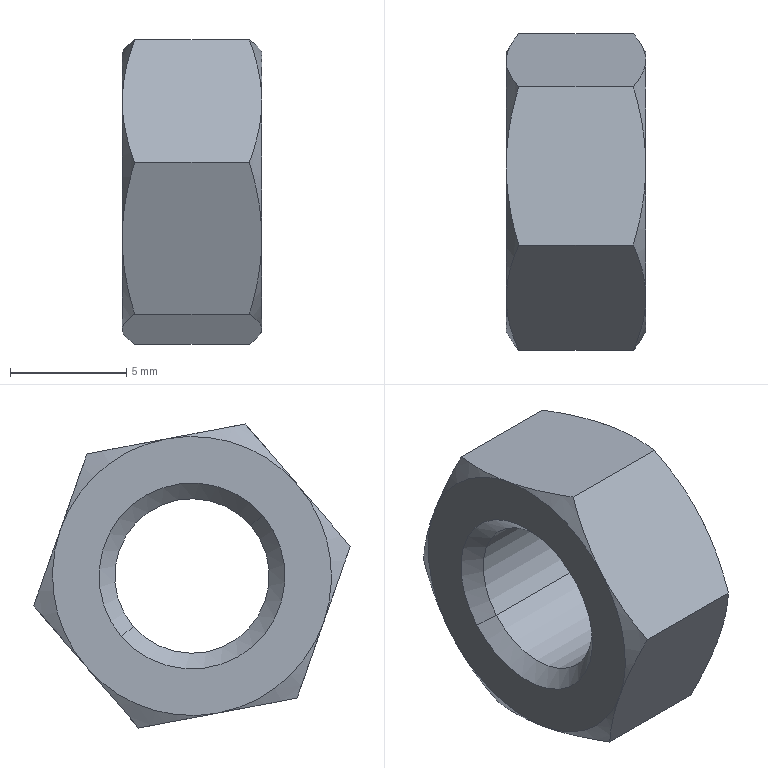Component | SolidWorks | CCDJSMA20x160SU(0)+(CS1-M-2)-1_CCDJS20 MA Nut1-1 | 1 solid | 26 faces | box 6 x 13.62 x 13.08 mm | volume 526 mm3 | cone 16 | plane 8 | cylinder 2 | commonest cylinder face diameters 6.647 x2
build123d program:
from build123d import *

# Parameters (mm, degrees)
CUT_EXTRUDE1_DEPTH      = 3
CUT_EXTRUDE1_DEPTH_BACK = 3
SKETCH3_W               = 24
SKETCH3_H               = 24


with BuildPart() as part:
    # Sketch1 → Revolve1 (revolve)
    with BuildSketch(Plane.XY, mode=Mode.PRIVATE) as revolve1_sk:
        Polygon((-3, 0), (-3, 6), (-2.307, 7.2), (2.307, 7.2), (3, 6), (3, 0), align=None)
    revolve(revolve1_sk.sketch.rotate(Axis((3, 0, 0), (-1, 0, 0)), 270), axis=Axis((3, 0, 0), (-1, 0, 0)))

    # Sketch2 → Cut-Revolve1 (revolve, cut)
    with BuildSketch(Plane.XY, mode=Mode.PRIVATE) as cut_revolve1_sk:
        Polygon((-3, 0), (-3, 4), (-2.324, 3.324), (2.324, 3.324), (3, 4), (3, 0), align=None)
    revolve(cut_revolve1_sk.sketch.rotate(Axis((3, 0, 0), (-1, 0, 0)), 270), axis=Axis((3, 0, 0), (-1, 0, 0)), mode=Mode.SUBTRACT)

    # Sketch3 → Cut-Extrude1 (cut, two sides: drawn at the far end of the back side and taken through both)
    with BuildSketch(Plane(origin=(0, 0, 0), x_dir=(0, 0, -1), z_dir=(1, 0, 0)).offset(-CUT_EXTRUDE1_DEPTH_BACK)):
        Rectangle(SKETCH3_W, SKETCH3_H)
        Polygon((-6, -3.464), (0, -6.928), (6, -3.464), (6, 3.464), (0, 6.928), (-6, 3.464), align=None, mode=Mode.SUBTRACT)
    extrude(amount=CUT_EXTRUDE1_DEPTH + CUT_EXTRUDE1_DEPTH_BACK, mode=Mode.SUBTRACT)


solid = part.part

# Placed as in the assembly
solid = solid.moved(Location((-82, 426.564, -63.57), (49.332, 0, 180)))
STEP:
#1=CARTESIAN_POINT('',(-3.32,16.695,-2.417));
#2=VERTEX_POINT('',#1);
#3=CARTESIAN_POINT('',(-3.32,16.893,-2.588));
#4=VERTEX_POINT('',#3);
#5=CARTESIAN_POINT('',(-3.32,16.794,-2.503));
#6=DIRECTION('',(1.,0.,0.));
#7=DIRECTION('',(0.,0.7584,-0.6518));
#8=AXIS2_PLACEMENT_3D('',#5,#6,#7);
#9=CIRCLE('',#8,0.1308);
#10=EDGE_CURVE('',#2,#4,#9,.T.);
#11=ORIENTED_EDGE('',*,*,#10,.T.);
#12=CARTESIAN_POINT('',(-3.346,16.913,-2.605));
#13=VERTEX_POINT('',#12);
#14=CARTESIAN_POINT('',(-3.346,16.913,-2.605));
#15=DIRECTION('',(-0.7071,0.5363,-0.4609));
#16=VECTOR('',#15,39.37);
#17=LINE('',#14,#16);
#18=EDGE_CURVE('',#4,#13,#17,.T.);
#19=ORIENTED_EDGE('',*,*,#18,.T.);
#20=CARTESIAN_POINT('',(-3.346,16.674,-2.4));
#21=VERTEX_POINT('',#20);
#22=CARTESIAN_POINT('',(-3.346,16.794,-2.503));
#23=DIRECTION('',(1.,0.,0.));
#24=DIRECTION('',(0.,0.7584,-0.6518));
#25=AXIS2_PLACEMENT_3D('',#22,#23,#24);
#26=CIRCLE('',#25,0.1575);
#27=EDGE_CURVE('',#21,#13,#26,.T.);
#28=ORIENTED_EDGE('',*,*,#27,.F.);
#29=CARTESIAN_POINT('',(-3.346,16.674,-2.4));
#30=DIRECTION('',(-0.7071,-0.5363,0.4609));
#31=VECTOR('',#30,39.37);
#32=LINE('',#29,#31);
#33=EDGE_CURVE('',#2,#21,#32,.T.);
#34=ORIENTED_EDGE('',*,*,#33,.F.);
#35=EDGE_LOOP('',(#11,#19,#28,#34));
#36=FACE_OUTER_BOUND('',#35,.T.);
#37=CARTESIAN_POINT('',(-3.346,16.794,-2.503));
#38=DIRECTION('',(-1.,0.,0.));
#39=DIRECTION('',(0.,-0.7584,0.6518));
#40=AXIS2_PLACEMENT_3D('',#37,#38,#39);
#41=CONICAL_SURFACE('',#40,0.1575,0.7854);
#42=ADVANCED_FACE('',(#36),#41,.F.);
#43=ORIENTED_EDGE('',*,*,#10,.F.);
#44=CARTESIAN_POINT('',(-3.137,16.695,-2.417));
#45=VERTEX_POINT('',#44);
#46=CARTESIAN_POINT('',(-3.346,16.695,-2.417));
#47=DIRECTION('',(1.,0.,0.));
#48=VECTOR('',#47,39.37);
#49=LINE('',#46,#48);
#50=EDGE_CURVE('',#2,#45,#49,.T.);
#51=ORIENTED_EDGE('',*,*,#50,.T.);
#52=CARTESIAN_POINT('',(-3.137,16.893,-2.588));
#53=VERTEX_POINT('',#52);
#54=CARTESIAN_POINT('',(-3.137,16.794,-2.503));
#55=DIRECTION('',(1.,0.,0.));
#56=DIRECTION('',(0.,0.7584,-0.6518));
#57=AXIS2_PLACEMENT_3D('',#54,#55,#56);
#58=CIRCLE('',#57,0.1308);
#59=EDGE_CURVE('',#45,#53,#58,.T.);
#60=ORIENTED_EDGE('',*,*,#59,.T.);
#61=CARTESIAN_POINT('',(-3.346,16.893,-2.588));
#62=DIRECTION('',(1.,0.,0.));
#63=VECTOR('',#62,39.37);
#64=LINE('',#61,#63);
#65=EDGE_CURVE('',#4,#53,#64,.T.);
#66=ORIENTED_EDGE('',*,*,#65,.F.);
#67=EDGE_LOOP('',(#43,#51,#60,#66));
#68=FACE_OUTER_BOUND('',#67,.T.);
#69=CARTESIAN_POINT('',(-3.346,16.794,-2.503));
#70=DIRECTION('',(1.,0.,0.));
#71=DIRECTION('',(0.,0.7584,-0.6518));
#72=AXIS2_PLACEMENT_3D('',#69,#70,#71);
#73=CYLINDRICAL_SURFACE('',#72,0.1308);
#74=ADVANCED_FACE('',(#68),#73,.F.);
#75=ORIENTED_EDGE('',*,*,#59,.F.);
#76=CARTESIAN_POINT('',(-3.11,16.674,-2.4));
#77=VERTEX_POINT('',#76);
#78=CARTESIAN_POINT('',(-3.137,16.695,-2.417));
#79=DIRECTION('',(0.7071,-0.5363,0.4609));
#80=VECTOR('',#79,39.37);
#81=LINE('',#78,#80);
#82=EDGE_CURVE('',#45,#77,#81,.T.);
#83=ORIENTED_EDGE('',*,*,#82,.T.);
#84=CARTESIAN_POINT('',(-3.11,16.913,-2.605));
#85=VERTEX_POINT('',#84);
#86=CARTESIAN_POINT('',(-3.11,16.794,-2.503));
#87=DIRECTION('',(1.,0.,0.));
#88=DIRECTION('',(0.,0.7584,-0.6518));
#89=AXIS2_PLACEMENT_3D('',#86,#87,#88);
#90=CIRCLE('',#89,0.1575);
#91=EDGE_CURVE('',#77,#85,#90,.T.);
#92=ORIENTED_EDGE('',*,*,#91,.T.);
#93=CARTESIAN_POINT('',(-3.137,16.893,-2.588));
#94=DIRECTION('',(0.7071,0.5363,-0.4609));
#95=VECTOR('',#94,39.37);
#96=LINE('',#93,#95);
#97=EDGE_CURVE('',#53,#85,#96,.T.);
#98=ORIENTED_EDGE('',*,*,#97,.F.);
#99=EDGE_LOOP('',(#75,#83,#92,#98));
#100=FACE_OUTER_BOUND('',#99,.T.);
#101=CARTESIAN_POINT('',(-3.137,16.794,-2.503));
#102=DIRECTION('',(1.,0.,0.));
#103=DIRECTION('',(0.,0.7584,-0.6518));
#104=AXIS2_PLACEMENT_3D('',#101,#102,#103);
#105=CONICAL_SURFACE('',#104,0.1308,0.7854);
#106=ADVANCED_FACE('',(#100),#105,.F.);
#107=CARTESIAN_POINT('',(-3.131,16.704,-2.245));
#108=VERTEX_POINT('',#107);
#109=CARTESIAN_POINT('',(-3.11,16.838,-2.271));
#110=VERTEX_POINT('',#109);
#111=CARTESIAN_POINT('',(-3.131,16.704,-2.245));
#112=CARTESIAN_POINT('',(-3.118,16.747,-2.254));
#113=CARTESIAN_POINT('',(-3.11,16.792,-2.262));
#114=CARTESIAN_POINT('',(-3.11,16.838,-2.271));
#115=B_SPLINE_CURVE_WITH_KNOTS('',3,(#111,#112,#113,#114),.UNSPECIFIED.,.F.,.F.,(4,4),(0.00000024,0.003505),.UNSPECIFIED.);
#116=EDGE_CURVE('',#108,#110,#115,.T.);
#117=ORIENTED_EDGE('',*,*,#116,.F.);
#118=CARTESIAN_POINT('',(-3.11,16.615,-2.349));
#119=VERTEX_POINT('',#118);
#120=CARTESIAN_POINT('',(-3.11,16.615,-2.349));
#121=CARTESIAN_POINT('',(-3.11,16.63,-2.331));
#122=CARTESIAN_POINT('',(-3.112,16.645,-2.314));
#123=CARTESIAN_POINT('',(-3.12,16.675,-2.279));
#124=CARTESIAN_POINT('',(-3.125,16.689,-2.262));
#125=CARTESIAN_POINT('',(-3.131,16.704,-2.245));
#126=B_SPLINE_CURVE_WITH_KNOTS('',3,(#120,#121,#122,#123,#124,#125),.UNSPECIFIED.,.F.,.F.,(4,2,4),(0.009709,0.01146,0.01322),.UNSPECIFIED.);
#127=EDGE_CURVE('',#119,#108,#126,.T.);
#128=ORIENTED_EDGE('',*,*,#127,.F.);
#129=CARTESIAN_POINT('',(-3.11,16.794,-2.503));
#130=DIRECTION('',(1.,0.,0.));
#131=DIRECTION('',(0.,0.7584,-0.6518));
#132=AXIS2_PLACEMENT_3D('',#129,#130,#131);
#133=CIRCLE('',#132,0.2362);
#134=EDGE_CURVE('',#110,#119,#133,.T.);
#135=ORIENTED_EDGE('',*,*,#134,.F.);
#136=EDGE_LOOP('',(#117,#128,#135));
#137=FACE_OUTER_BOUND('',#136,.T.);
#138=CARTESIAN_POINT('',(-3.138,16.794,-2.503));
#139=DIRECTION('',(-1.,0.,0.));
#140=DIRECTION('',(0.,-0.7584,0.6518));
#141=AXIS2_PLACEMENT_3D('',#138,#139,#140);
#142=CONICAL_SURFACE('',#141,0.2835,1.047);
#143=ADVANCED_FACE('',(#137),#142,.T.);
#144=CARTESIAN_POINT('',(-3.131,16.972,-2.296));
#145=VERTEX_POINT('',#144);
#146=CARTESIAN_POINT('',(-3.11,16.838,-2.271));
#147=CARTESIAN_POINT('',(-3.11,16.849,-2.273));
#148=CARTESIAN_POINT('',(-3.111,16.86,-2.275));
#149=CARTESIAN_POINT('',(-3.113,16.883,-2.279));
#150=CARTESIAN_POINT('',(-3.114,16.894,-2.281));
#151=CARTESIAN_POINT('',(-3.12,16.928,-2.288));
#152=CARTESIAN_POINT('',(-3.125,16.95,-2.292));
#153=CARTESIAN_POINT('',(-3.131,16.972,-2.296));
#154=B_SPLINE_CURVE_WITH_KNOTS('',3,(#146,#147,#148,#149,#150,#151,#152,#153),.UNSPECIFIED.,.F.,.F.,(4,2,2,4),(0.003505,0.004378,0.005251,0.006997),.UNSPECIFIED.);
#155=EDGE_CURVE('',#110,#145,#154,.T.);
#156=ORIENTED_EDGE('',*,*,#155,.F.);
#157=CARTESIAN_POINT('',(-3.11,17.017,-2.425));
#158=VERTEX_POINT('',#157);
#159=CARTESIAN_POINT('',(-3.11,16.794,-2.503));
#160=DIRECTION('',(1.,0.,0.));
#161=DIRECTION('',(0.,0.7584,-0.6518));
#162=AXIS2_PLACEMENT_3D('',#159,#160,#161);
#163=CIRCLE('',#162,0.2362);
#164=EDGE_CURVE('',#158,#110,#163,.T.);
#165=ORIENTED_EDGE('',*,*,#164,.F.);
#166=CARTESIAN_POINT('',(-3.131,16.972,-2.296));
#167=CARTESIAN_POINT('',(-3.118,16.986,-2.338));
#168=CARTESIAN_POINT('',(-3.11,17.001,-2.381));
#169=CARTESIAN_POINT('',(-3.11,17.017,-2.425));
#170=B_SPLINE_CURVE_WITH_KNOTS('',3,(#166,#167,#168,#169),.UNSPECIFIED.,.F.,.F.,(4,4),(0.00000024,0.003505),.UNSPECIFIED.);
#171=EDGE_CURVE('',#145,#158,#170,.T.);
#172=ORIENTED_EDGE('',*,*,#171,.F.);
#173=EDGE_LOOP('',(#156,#165,#172));
#174=FACE_OUTER_BOUND('',#173,.T.);
#175=CARTESIAN_POINT('',(-3.138,16.794,-2.503));
#176=DIRECTION('',(-1.,0.,0.));
#177=DIRECTION('',(0.,-0.7584,0.6518));
#178=AXIS2_PLACEMENT_3D('',#175,#176,#177);
#179=CONICAL_SURFACE('',#178,0.2835,1.047);
#180=ADVANCED_FACE('',(#174),#179,.T.);
#181=CARTESIAN_POINT('',(-3.131,17.062,-2.553));
#182=VERTEX_POINT('',#181);
#183=CARTESIAN_POINT('',(-3.11,17.017,-2.425));
#184=CARTESIAN_POINT('',(-3.11,17.021,-2.436));
#185=CARTESIAN_POINT('',(-3.111,17.024,-2.446));
#186=CARTESIAN_POINT('',(-3.113,17.032,-2.468));
#187=CARTESIAN_POINT('',(-3.114,17.036,-2.479));
#188=CARTESIAN_POINT('',(-3.12,17.047,-2.511));
#189=CARTESIAN_POINT('',(-3.125,17.055,-2.532));
#190=CARTESIAN_POINT('',(-3.131,17.062,-2.553));
#191=B_SPLINE_CURVE_WITH_KNOTS('',3,(#183,#184,#185,#186,#187,#188,#189,#190),.UNSPECIFIED.,.F.,.F.,(4,2,2,4),(0.003505,0.004378,0.005251,0.006997),.UNSPECIFIED.);
#192=EDGE_CURVE('',#158,#182,#191,.T.);
#193=ORIENTED_EDGE('',*,*,#192,.F.);
#194=CARTESIAN_POINT('',(-3.11,16.973,-2.657));
#195=VERTEX_POINT('',#194);
#196=CARTESIAN_POINT('',(-3.11,16.794,-2.503));
#197=DIRECTION('',(1.,0.,0.));
#198=DIRECTION('',(0.,0.7584,-0.6518));
#199=AXIS2_PLACEMENT_3D('',#196,#197,#198);
#200=CIRCLE('',#199,0.2362);
#201=EDGE_CURVE('',#195,#158,#200,.T.);
#202=ORIENTED_EDGE('',*,*,#201,.F.);
#203=CARTESIAN_POINT('',(-3.131,17.062,-2.553));
#204=CARTESIAN_POINT('',(-3.125,17.048,-2.57));
#205=CARTESIAN_POINT('',(-3.12,17.033,-2.587));
#206=CARTESIAN_POINT('',(-3.112,17.003,-2.622));
#207=CARTESIAN_POINT('',(-3.11,16.988,-2.639));
#208=CARTESIAN_POINT('',(-3.11,16.973,-2.657));
#209=B_SPLINE_CURVE_WITH_KNOTS('',3,(#203,#204,#205,#206,#207,#208),.UNSPECIFIED.,.F.,.F.,(4,2,4),(0.01521,0.01696,0.01872),.UNSPECIFIED.);
#210=EDGE_CURVE('',#182,#195,#209,.T.);
#211=ORIENTED_EDGE('',*,*,#210,.F.);
#212=EDGE_LOOP('',(#193,#202,#211));
#213=FACE_OUTER_BOUND('',#212,.T.);
#214=CARTESIAN_POINT('',(-3.138,16.794,-2.503));
#215=DIRECTION('',(-1.,0.,0.));
#216=DIRECTION('',(0.,-0.7584,0.6518));
#217=AXIS2_PLACEMENT_3D('',#214,#215,#216);
#218=CONICAL_SURFACE('',#217,0.2835,1.047);
#219=ADVANCED_FACE('',(#213),#218,.T.);
#220=CARTESIAN_POINT('',(-3.131,16.526,-2.452));
#221=VERTEX_POINT('',#220);
#222=CARTESIAN_POINT('',(-3.131,16.526,-2.452));
#223=CARTESIAN_POINT('',(-3.125,16.54,-2.435));
#224=CARTESIAN_POINT('',(-3.12,16.555,-2.418));
#225=CARTESIAN_POINT('',(-3.112,16.585,-2.384));
#226=CARTESIAN_POINT('',(-3.11,16.6,-2.366));
#227=CARTESIAN_POINT('',(-3.11,16.615,-2.349));
#228=B_SPLINE_CURVE_WITH_KNOTS('',3,(#222,#223,#224,#225,#226,#227),.UNSPECIFIED.,.F.,.F.,(4,2,4),(0.006205,0.007957,0.009709),.UNSPECIFIED.);
#229=EDGE_CURVE('',#221,#119,#228,.T.);
#230=ORIENTED_EDGE('',*,*,#229,.F.);
#231=CARTESIAN_POINT('',(-3.11,16.571,-2.581));
#232=VERTEX_POINT('',#231);
#233=CARTESIAN_POINT('',(-3.11,16.571,-2.581));
#234=CARTESIAN_POINT('',(-3.11,16.567,-2.57));
#235=CARTESIAN_POINT('',(-3.111,16.563,-2.559));
#236=CARTESIAN_POINT('',(-3.113,16.556,-2.537));
#237=CARTESIAN_POINT('',(-3.114,16.552,-2.527));
#238=CARTESIAN_POINT('',(-3.12,16.541,-2.494));
#239=CARTESIAN_POINT('',(-3.125,16.533,-2.473));
#240=CARTESIAN_POINT('',(-3.131,16.526,-2.452));
#241=B_SPLINE_CURVE_WITH_KNOTS('',3,(#233,#234,#235,#236,#237,#238,#239,#240),.UNSPECIFIED.,.F.,.F.,(4,2,2,4),(0.003505,0.004378,0.005251,0.006997),.UNSPECIFIED.);
#242=EDGE_CURVE('',#232,#221,#241,.T.);
#243=ORIENTED_EDGE('',*,*,#242,.F.);
#244=CARTESIAN_POINT('',(-3.11,16.794,-2.503));
#245=DIRECTION('',(1.,0.,0.));
#246=DIRECTION('',(0.,0.7584,-0.6518));
#247=AXIS2_PLACEMENT_3D('',#244,#245,#246);
#248=CIRCLE('',#247,0.2362);
#249=EDGE_CURVE('',#119,#232,#248,.T.);
#250=ORIENTED_EDGE('',*,*,#249,.F.);
#251=EDGE_LOOP('',(#230,#243,#250));
#252=FACE_OUTER_BOUND('',#251,.T.);
#253=CARTESIAN_POINT('',(-3.138,16.794,-2.503));
#254=DIRECTION('',(-1.,0.,0.));
#255=DIRECTION('',(0.,-0.7584,0.6518));
#256=AXIS2_PLACEMENT_3D('',#253,#254,#255);
#257=CONICAL_SURFACE('',#256,0.2835,1.047);
#258=ADVANCED_FACE('',(#252),#257,.T.);
#259=CARTESIAN_POINT('',(-3.131,16.884,-2.76));
#260=VERTEX_POINT('',#259);
#261=CARTESIAN_POINT('',(-3.11,16.973,-2.657));
#262=CARTESIAN_POINT('',(-3.11,16.958,-2.674));
#263=CARTESIAN_POINT('',(-3.112,16.943,-2.692));
#264=CARTESIAN_POINT('',(-3.12,16.913,-2.726));
#265=CARTESIAN_POINT('',(-3.125,16.899,-2.743));
#266=CARTESIAN_POINT('',(-3.131,16.884,-2.76));
#267=B_SPLINE_CURVE_WITH_KNOTS('',3,(#261,#262,#263,#264,#265,#266),.UNSPECIFIED.,.F.,.F.,(4,2,4),(0.01872,0.02047,0.02223),.UNSPECIFIED.);
#268=EDGE_CURVE('',#195,#260,#267,.T.);
#269=ORIENTED_EDGE('',*,*,#268,.F.);
#270=CARTESIAN_POINT('',(-3.11,16.75,-2.735));
#271=VERTEX_POINT('',#270);
#272=CARTESIAN_POINT('',(-3.11,16.794,-2.503));
#273=DIRECTION('',(1.,0.,0.));
#274=DIRECTION('',(0.,0.7584,-0.6518));
#275=AXIS2_PLACEMENT_3D('',#272,#273,#274);
#276=CIRCLE('',#275,0.2362);
#277=EDGE_CURVE('',#271,#195,#276,.T.);
#278=ORIENTED_EDGE('',*,*,#277,.F.);
#279=CARTESIAN_POINT('',(-3.131,16.884,-2.76));
#280=CARTESIAN_POINT('',(-3.118,16.84,-2.752));
#281=CARTESIAN_POINT('',(-3.11,16.796,-2.743));
#282=CARTESIAN_POINT('',(-3.11,16.75,-2.735));
#283=B_SPLINE_CURVE_WITH_KNOTS('',3,(#279,#280,#281,#282),.UNSPECIFIED.,.F.,.F.,(4,4),(0.00000024,0.003505),.UNSPECIFIED.);
#284=EDGE_CURVE('',#260,#271,#283,.T.);
#285=ORIENTED_EDGE('',*,*,#284,.F.);
#286=EDGE_LOOP('',(#269,#278,#285));
#287=FACE_OUTER_BOUND('',#286,.T.);
#288=CARTESIAN_POINT('',(-3.138,16.794,-2.503));
#289=DIRECTION('',(-1.,0.,0.));
#290=DIRECTION('',(0.,-0.7584,0.6518));
#291=AXIS2_PLACEMENT_3D('',#288,#289,#290);
#292=CONICAL_SURFACE('',#291,0.2835,1.047);
#293=ADVANCED_FACE('',(#287),#292,.T.);
#294=CARTESIAN_POINT('',(-3.131,16.616,-2.71));
#295=VERTEX_POINT('',#294);
#296=CARTESIAN_POINT('',(-3.131,16.616,-2.71));
#297=CARTESIAN_POINT('',(-3.118,16.601,-2.668));
#298=CARTESIAN_POINT('',(-3.11,16.586,-2.625));
#299=CARTESIAN_POINT('',(-3.11,16.571,-2.581));
#300=B_SPLINE_CURVE_WITH_KNOTS('',3,(#296,#297,#298,#299),.UNSPECIFIED.,.F.,.F.,(4,4),(0.00000024,0.003505),.UNSPECIFIED.);
#301=EDGE_CURVE('',#295,#232,#300,.T.);
#302=ORIENTED_EDGE('',*,*,#301,.F.);
#303=CARTESIAN_POINT('',(-3.11,16.75,-2.735));
#304=CARTESIAN_POINT('',(-3.11,16.739,-2.733));
#305=CARTESIAN_POINT('',(-3.111,16.727,-2.731));
#306=CARTESIAN_POINT('',(-3.113,16.705,-2.726));
#307=CARTESIAN_POINT('',(-3.114,16.693,-2.724));
#308=CARTESIAN_POINT('',(-3.12,16.66,-2.718));
#309=CARTESIAN_POINT('',(-3.125,16.638,-2.714));
#310=CARTESIAN_POINT('',(-3.131,16.616,-2.71));
#311=B_SPLINE_CURVE_WITH_KNOTS('',3,(#303,#304,#305,#306,#307,#308,#309,#310),.UNSPECIFIED.,.F.,.F.,(4,2,2,4),(0.003505,0.004378,0.005251,0.006997),.UNSPECIFIED.);
#312=EDGE_CURVE('',#271,#295,#311,.T.);
#313=ORIENTED_EDGE('',*,*,#312,.F.);
#314=CARTESIAN_POINT('',(-3.11,16.794,-2.503));
#315=DIRECTION('',(1.,0.,0.));
#316=DIRECTION('',(0.,0.7584,-0.6518));
#317=AXIS2_PLACEMENT_3D('',#314,#315,#316);
#318=CIRCLE('',#317,0.2362);
#319=EDGE_CURVE('',#232,#271,#318,.T.);
#320=ORIENTED_EDGE('',*,*,#319,.F.);
#321=EDGE_LOOP('',(#302,#313,#320));
#322=FACE_OUTER_BOUND('',#321,.T.);
#323=CARTESIAN_POINT('',(-3.138,16.794,-2.503));
#324=DIRECTION('',(-1.,0.,0.));
#325=DIRECTION('',(0.,-0.7584,0.6518));
#326=AXIS2_PLACEMENT_3D('',#323,#324,#325);
#327=CONICAL_SURFACE('',#326,0.2835,1.047);
#328=ADVANCED_FACE('',(#322),#327,.T.);
#329=CARTESIAN_POINT('',(-3.325,16.884,-2.76));
#330=VERTEX_POINT('',#329);
#331=CARTESIAN_POINT('',(-3.346,16.973,-2.657));
#332=VERTEX_POINT('',#331);
#333=CARTESIAN_POINT('',(-3.325,16.884,-2.76));
#334=CARTESIAN_POINT('',(-3.332,16.899,-2.743));
#335=CARTESIAN_POINT('',(-3.337,16.913,-2.726));
#336=CARTESIAN_POINT('',(-3.344,16.943,-2.692));
#337=CARTESIAN_POINT('',(-3.346,16.958,-2.674));
#338=CARTESIAN_POINT('',(-3.346,16.973,-2.657));
#339=B_SPLINE_CURVE_WITH_KNOTS('',3,(#333,#334,#335,#336,#337,#338),.UNSPECIFIED.,.F.,.F.,(4,2,4),(0.006205,0.007957,0.009709),.UNSPECIFIED.);
#340=EDGE_CURVE('',#330,#332,#339,.T.);
#341=ORIENTED_EDGE('',*,*,#340,.F.);
#342=CARTESIAN_POINT('',(-3.346,16.75,-2.735));
#343=VERTEX_POINT('',#342);
#344=CARTESIAN_POINT('',(-3.346,16.75,-2.735));
#345=CARTESIAN_POINT('',(-3.346,16.761,-2.737));
#346=CARTESIAN_POINT('',(-3.346,16.773,-2.739));
#347=CARTESIAN_POINT('',(-3.344,16.796,-2.743));
#348=CARTESIAN_POINT('',(-3.343,16.807,-2.746));
#349=CARTESIAN_POINT('',(-3.337,16.84,-2.752));
#350=CARTESIAN_POINT('',(-3.332,16.862,-2.756));
#351=CARTESIAN_POINT('',(-3.325,16.884,-2.76));
#352=B_SPLINE_CURVE_WITH_KNOTS('',3,(#344,#345,#346,#347,#348,#349,#350,#351),.UNSPECIFIED.,.F.,.F.,(4,2,2,4),(0.003505,0.004378,0.005251,0.006997),.UNSPECIFIED.);
#353=EDGE_CURVE('',#343,#330,#352,.T.);
#354=ORIENTED_EDGE('',*,*,#353,.F.);
#355=CARTESIAN_POINT('',(-3.346,16.794,-2.503));
#356=DIRECTION('',(1.,0.,0.));
#357=DIRECTION('',(0.,0.7584,-0.6518));
#358=AXIS2_PLACEMENT_3D('',#355,#356,#357);
#359=CIRCLE('',#358,0.2362);
#360=EDGE_CURVE('',#343,#332,#359,.T.);
#361=ORIENTED_EDGE('',*,*,#360,.T.);
#362=EDGE_LOOP('',(#341,#354,#361));
#363=FACE_OUTER_BOUND('',#362,.T.);
#364=CARTESIAN_POINT('',(-3.346,16.794,-2.503));
#365=DIRECTION('',(1.,0.,0.));
#366=DIRECTION('',(0.,0.7584,-0.6518));
#367=AXIS2_PLACEMENT_3D('',#364,#365,#366);
#368=CONICAL_SURFACE('',#367,0.2362,1.047);
#369=ADVANCED_FACE('',(#363),#368,.T.);
#370=CARTESIAN_POINT('',(-3.325,17.062,-2.553));
#371=VERTEX_POINT('',#370);
#372=CARTESIAN_POINT('',(-3.346,16.973,-2.657));
#373=CARTESIAN_POINT('',(-3.346,16.988,-2.639));
#374=CARTESIAN_POINT('',(-3.344,17.003,-2.622));
#375=CARTESIAN_POINT('',(-3.337,17.033,-2.587));
#376=CARTESIAN_POINT('',(-3.332,17.048,-2.57));
#377=CARTESIAN_POINT('',(-3.325,17.062,-2.553));
#378=B_SPLINE_CURVE_WITH_KNOTS('',3,(#372,#373,#374,#375,#376,#377),.UNSPECIFIED.,.F.,.F.,(4,2,4),(0.009709,0.01146,0.01322),.UNSPECIFIED.);
#379=EDGE_CURVE('',#332,#371,#378,.T.);
#380=ORIENTED_EDGE('',*,*,#379,.F.);
#381=CARTESIAN_POINT('',(-3.346,17.017,-2.425));
#382=VERTEX_POINT('',#381);
#383=CARTESIAN_POINT('',(-3.346,16.794,-2.503));
#384=DIRECTION('',(1.,0.,0.));
#385=DIRECTION('',(0.,0.7584,-0.6518));
#386=AXIS2_PLACEMENT_3D('',#383,#384,#385);
#387=CIRCLE('',#386,0.2362);
#388=EDGE_CURVE('',#332,#382,#387,.T.);
#389=ORIENTED_EDGE('',*,*,#388,.T.);
#390=CARTESIAN_POINT('',(-3.325,17.062,-2.553));
#391=CARTESIAN_POINT('',(-3.338,17.047,-2.511));
#392=CARTESIAN_POINT('',(-3.346,17.032,-2.468));
#393=CARTESIAN_POINT('',(-3.346,17.017,-2.425));
#394=B_SPLINE_CURVE_WITH_KNOTS('',3,(#390,#391,#392,#393),.UNSPECIFIED.,.F.,.F.,(4,4),(0.00000024,0.003505),.UNSPECIFIED.);
#395=EDGE_CURVE('',#371,#382,#394,.T.);
#396=ORIENTED_EDGE('',*,*,#395,.F.);
#397=EDGE_LOOP('',(#380,#389,#396));
#398=FACE_OUTER_BOUND('',#397,.T.);
#399=CARTESIAN_POINT('',(-3.346,16.794,-2.503));
#400=DIRECTION('',(1.,0.,0.));
#401=DIRECTION('',(0.,0.7584,-0.6518));
#402=AXIS2_PLACEMENT_3D('',#399,#400,#401);
#403=CONICAL_SURFACE('',#402,0.2362,1.047);
#404=ADVANCED_FACE('',(#398),#403,.T.);
#405=CARTESIAN_POINT('',(-3.325,16.972,-2.296));
#406=VERTEX_POINT('',#405);
#407=CARTESIAN_POINT('',(-3.346,17.017,-2.425));
#408=CARTESIAN_POINT('',(-3.346,17.013,-2.414));
#409=CARTESIAN_POINT('',(-3.346,17.009,-2.403));
#410=CARTESIAN_POINT('',(-3.344,17.002,-2.381));
#411=CARTESIAN_POINT('',(-3.343,16.998,-2.37));
#412=CARTESIAN_POINT('',(-3.337,16.986,-2.338));
#413=CARTESIAN_POINT('',(-3.332,16.979,-2.317));
#414=CARTESIAN_POINT('',(-3.325,16.972,-2.296));
#415=B_SPLINE_CURVE_WITH_KNOTS('',3,(#407,#408,#409,#410,#411,#412,#413,#414),.UNSPECIFIED.,.F.,.F.,(4,2,2,4),(0.003505,0.004378,0.005251,0.006997),.UNSPECIFIED.);
#416=EDGE_CURVE('',#382,#406,#415,.T.);
#417=ORIENTED_EDGE('',*,*,#416,.F.);
#418=CARTESIAN_POINT('',(-3.346,16.838,-2.271));
#419=VERTEX_POINT('',#418);
#420=CARTESIAN_POINT('',(-3.346,16.794,-2.503));
#421=DIRECTION('',(1.,0.,0.));
#422=DIRECTION('',(0.,0.7584,-0.6518));
#423=AXIS2_PLACEMENT_3D('',#420,#421,#422);
#424=CIRCLE('',#423,0.2362);
#425=EDGE_CURVE('',#382,#419,#424,.T.);
#426=ORIENTED_EDGE('',*,*,#425,.T.);
#427=CARTESIAN_POINT('',(-3.325,16.972,-2.296));
#428=CARTESIAN_POINT('',(-3.338,16.928,-2.288));
#429=CARTESIAN_POINT('',(-3.346,16.883,-2.279));
#430=CARTESIAN_POINT('',(-3.346,16.838,-2.271));
#431=B_SPLINE_CURVE_WITH_KNOTS('',3,(#427,#428,#429,#430),.UNSPECIFIED.,.F.,.F.,(4,4),(0.00000024,0.003505),.UNSPECIFIED.);
#432=EDGE_CURVE('',#406,#419,#431,.T.);
#433=ORIENTED_EDGE('',*,*,#432,.F.);
#434=EDGE_LOOP('',(#417,#426,#433));
#435=FACE_OUTER_BOUND('',#434,.T.);
#436=CARTESIAN_POINT('',(-3.346,16.794,-2.503));
#437=DIRECTION('',(1.,0.,0.));
#438=DIRECTION('',(0.,0.7584,-0.6518));
#439=AXIS2_PLACEMENT_3D('',#436,#437,#438);
#440=CONICAL_SURFACE('',#439,0.2362,1.047);
#441=ADVANCED_FACE('',(#435),#440,.T.);
#442=CARTESIAN_POINT('',(-3.325,16.704,-2.245));
#443=VERTEX_POINT('',#442);
#444=CARTESIAN_POINT('',(-3.346,16.838,-2.271));
#445=CARTESIAN_POINT('',(-3.346,16.826,-2.268));
#446=CARTESIAN_POINT('',(-3.346,16.815,-2.266));
#447=CARTESIAN_POINT('',(-3.344,16.792,-2.262));
#448=CARTESIAN_POINT('',(-3.343,16.781,-2.26));
#449=CARTESIAN_POINT('',(-3.337,16.748,-2.254));
#450=CARTESIAN_POINT('',(-3.332,16.725,-2.249));
#451=CARTESIAN_POINT('',(-3.325,16.704,-2.245));
#452=B_SPLINE_CURVE_WITH_KNOTS('',3,(#444,#445,#446,#447,#448,#449,#450,#451),.UNSPECIFIED.,.F.,.F.,(4,2,2,4),(0.003505,0.004378,0.005251,0.006997),.UNSPECIFIED.);
#453=EDGE_CURVE('',#419,#443,#452,.T.);
#454=ORIENTED_EDGE('',*,*,#453,.F.);
#455=CARTESIAN_POINT('',(-3.346,16.615,-2.349));
#456=VERTEX_POINT('',#455);
#457=CARTESIAN_POINT('',(-3.346,16.794,-2.503));
#458=DIRECTION('',(1.,0.,0.));
#459=DIRECTION('',(0.,0.7584,-0.6518));
#460=AXIS2_PLACEMENT_3D('',#457,#458,#459);
#461=CIRCLE('',#460,0.2362);
#462=EDGE_CURVE('',#419,#456,#461,.T.);
#463=ORIENTED_EDGE('',*,*,#462,.T.);
#464=CARTESIAN_POINT('',(-3.325,16.704,-2.245));
#465=CARTESIAN_POINT('',(-3.332,16.689,-2.262));
#466=CARTESIAN_POINT('',(-3.337,16.675,-2.279));
#467=CARTESIAN_POINT('',(-3.344,16.645,-2.314));
#468=CARTESIAN_POINT('',(-3.346,16.63,-2.331));
#469=CARTESIAN_POINT('',(-3.346,16.615,-2.349));
#470=B_SPLINE_CURVE_WITH_KNOTS('',3,(#464,#465,#466,#467,#468,#469),.UNSPECIFIED.,.F.,.F.,(4,2,4),(0.01521,0.01696,0.01872),.UNSPECIFIED.);
#471=EDGE_CURVE('',#443,#456,#470,.T.);
#472=ORIENTED_EDGE('',*,*,#471,.F.);
#473=EDGE_LOOP('',(#454,#463,#472));
#474=FACE_OUTER_BOUND('',#473,.T.);
#475=CARTESIAN_POINT('',(-3.346,16.794,-2.503));
#476=DIRECTION('',(1.,0.,0.));
#477=DIRECTION('',(0.,0.7584,-0.6518));
#478=AXIS2_PLACEMENT_3D('',#475,#476,#477);
#479=CONICAL_SURFACE('',#478,0.2362,1.047);
#480=ADVANCED_FACE('',(#474),#479,.T.);
#481=CARTESIAN_POINT('',(-3.325,16.526,-2.452));
#482=VERTEX_POINT('',#481);
#483=CARTESIAN_POINT('',(-3.346,16.615,-2.349));
#484=CARTESIAN_POINT('',(-3.346,16.6,-2.366));
#485=CARTESIAN_POINT('',(-3.344,16.585,-2.384));
#486=CARTESIAN_POINT('',(-3.337,16.555,-2.418));
#487=CARTESIAN_POINT('',(-3.332,16.54,-2.435));
#488=CARTESIAN_POINT('',(-3.325,16.526,-2.452));
#489=B_SPLINE_CURVE_WITH_KNOTS('',3,(#483,#484,#485,#486,#487,#488),.UNSPECIFIED.,.F.,.F.,(4,2,4),(0.01872,0.02047,0.02223),.UNSPECIFIED.);
#490=EDGE_CURVE('',#456,#482,#489,.T.);
#491=ORIENTED_EDGE('',*,*,#490,.F.);
#492=CARTESIAN_POINT('',(-3.346,16.571,-2.581));
#493=VERTEX_POINT('',#492);
#494=CARTESIAN_POINT('',(-3.346,16.794,-2.503));
#495=DIRECTION('',(1.,0.,0.));
#496=DIRECTION('',(0.,0.7584,-0.6518));
#497=AXIS2_PLACEMENT_3D('',#494,#495,#496);
#498=CIRCLE('',#497,0.2362);
#499=EDGE_CURVE('',#456,#493,#498,.T.);
#500=ORIENTED_EDGE('',*,*,#499,.T.);
#501=CARTESIAN_POINT('',(-3.325,16.526,-2.452));
#502=CARTESIAN_POINT('',(-3.338,16.541,-2.494));
#503=CARTESIAN_POINT('',(-3.346,16.556,-2.537));
#504=CARTESIAN_POINT('',(-3.346,16.571,-2.581));
#505=B_SPLINE_CURVE_WITH_KNOTS('',3,(#501,#502,#503,#504),.UNSPECIFIED.,.F.,.F.,(4,4),(0.00000024,0.003505),.UNSPECIFIED.);
#506=EDGE_CURVE('',#482,#493,#505,.T.);
#507=ORIENTED_EDGE('',*,*,#506,.F.);
#508=EDGE_LOOP('',(#491,#500,#507));
#509=FACE_OUTER_BOUND('',#508,.T.);
#510=CARTESIAN_POINT('',(-3.346,16.794,-2.503));
#511=DIRECTION('',(1.,0.,0.));
#512=DIRECTION('',(0.,0.7584,-0.6518));
#513=AXIS2_PLACEMENT_3D('',#510,#511,#512);
#514=CONICAL_SURFACE('',#513,0.2362,1.047);
#515=ADVANCED_FACE('',(#509),#514,.T.);
#516=CARTESIAN_POINT('',(-3.325,16.616,-2.71));
#517=VERTEX_POINT('',#516);
#518=CARTESIAN_POINT('',(-3.346,16.571,-2.581));
#519=CARTESIAN_POINT('',(-3.346,16.575,-2.592));
#520=CARTESIAN_POINT('',(-3.346,16.579,-2.603));
#521=CARTESIAN_POINT('',(-3.344,16.586,-2.625));
#522=CARTESIAN_POINT('',(-3.343,16.59,-2.635));
#523=CARTESIAN_POINT('',(-3.337,16.601,-2.667));
#524=CARTESIAN_POINT('',(-3.332,16.609,-2.689));
#525=CARTESIAN_POINT('',(-3.325,16.616,-2.71));
#526=B_SPLINE_CURVE_WITH_KNOTS('',3,(#518,#519,#520,#521,#522,#523,#524,#525),.UNSPECIFIED.,.F.,.F.,(4,2,2,4),(0.003505,0.004378,0.005251,0.006997),.UNSPECIFIED.);
#527=EDGE_CURVE('',#493,#517,#526,.T.);
#528=ORIENTED_EDGE('',*,*,#527,.F.);
#529=CARTESIAN_POINT('',(-3.346,16.794,-2.503));
#530=DIRECTION('',(1.,0.,0.));
#531=DIRECTION('',(0.,0.7584,-0.6518));
#532=AXIS2_PLACEMENT_3D('',#529,#530,#531);
#533=CIRCLE('',#532,0.2362);
#534=EDGE_CURVE('',#493,#343,#533,.T.);
#535=ORIENTED_EDGE('',*,*,#534,.T.);
#536=CARTESIAN_POINT('',(-3.325,16.616,-2.71));
#537=CARTESIAN_POINT('',(-3.338,16.66,-2.718));
#538=CARTESIAN_POINT('',(-3.346,16.704,-2.726));
#539=CARTESIAN_POINT('',(-3.346,16.75,-2.735));
#540=B_SPLINE_CURVE_WITH_KNOTS('',3,(#536,#537,#538,#539),.UNSPECIFIED.,.F.,.F.,(4,4),(0.00000024,0.003505),.UNSPECIFIED.);
#541=EDGE_CURVE('',#517,#343,#540,.T.);
#542=ORIENTED_EDGE('',*,*,#541,.F.);
#543=EDGE_LOOP('',(#528,#535,#542));
#544=FACE_OUTER_BOUND('',#543,.T.);
#545=CARTESIAN_POINT('',(-3.346,16.794,-2.503));
#546=DIRECTION('',(1.,0.,0.));
#547=DIRECTION('',(0.,0.7584,-0.6518));
#548=AXIS2_PLACEMENT_3D('',#545,#546,#547);
#549=CONICAL_SURFACE('',#548,0.2362,1.047);
#550=ADVANCED_FACE('',(#544),#549,.T.);
#551=CARTESIAN_POINT('',(-3.11,16.794,-2.503));
#552=DIRECTION('',(1.,0.,0.));
#553=DIRECTION('',(0.,0.7584,-0.6518));
#554=AXIS2_PLACEMENT_3D('',#551,#552,#553);
#555=CIRCLE('',#554,0.1575);
#556=EDGE_CURVE('',#85,#77,#555,.T.);
#557=ORIENTED_EDGE('',*,*,#556,.F.);
#558=ORIENTED_EDGE('',*,*,#91,.F.);
#559=EDGE_LOOP('',(#557,#558));
#560=FACE_BOUND('',#559,.T.);
#561=ORIENTED_EDGE('',*,*,#201,.T.);
#562=ORIENTED_EDGE('',*,*,#164,.T.);
#563=ORIENTED_EDGE('',*,*,#134,.T.);
#564=ORIENTED_EDGE('',*,*,#249,.T.);
#565=ORIENTED_EDGE('',*,*,#319,.T.);
#566=ORIENTED_EDGE('',*,*,#277,.T.);
#567=EDGE_LOOP('',(#561,#562,#563,#564,#565,#566));
#568=FACE_OUTER_BOUND('',#567,.T.);
#569=CARTESIAN_POINT('',(-3.11,16.794,-2.503));
#570=DIRECTION('',(-1.,0.,0.));
#571=DIRECTION('',(0.,-0.7584,0.6518));
#572=AXIS2_PLACEMENT_3D('',#569,#570,#571);
#573=PLANE('',#572);
#574=ADVANCED_FACE('',(#560,#568),#573,.F.);
#575=ORIENTED_EDGE('',*,*,#27,.T.);
#576=CARTESIAN_POINT('',(-3.346,16.794,-2.503));
#577=DIRECTION('',(1.,0.,0.));
#578=DIRECTION('',(0.,0.7584,-0.6518));
#579=AXIS2_PLACEMENT_3D('',#576,#577,#578);
#580=CIRCLE('',#579,0.1575);
#581=EDGE_CURVE('',#13,#21,#580,.T.);
#582=ORIENTED_EDGE('',*,*,#581,.T.);
#583=EDGE_LOOP('',(#575,#582));
#584=FACE_BOUND('',#583,.T.);
#585=ORIENTED_EDGE('',*,*,#388,.F.);
#586=ORIENTED_EDGE('',*,*,#360,.F.);
#587=ORIENTED_EDGE('',*,*,#534,.F.);
#588=ORIENTED_EDGE('',*,*,#499,.F.);
#589=ORIENTED_EDGE('',*,*,#462,.F.);
#590=ORIENTED_EDGE('',*,*,#425,.F.);
#591=EDGE_LOOP('',(#585,#586,#587,#588,#589,#590));
#592=FACE_OUTER_BOUND('',#591,.T.);
#593=CARTESIAN_POINT('',(-3.346,16.948,-2.324));
#594=DIRECTION('',(1.,0.,0.));
#595=DIRECTION('',(0.,0.7584,-0.6518));
#596=AXIS2_PLACEMENT_3D('',#593,#594,#595);
#597=PLANE('',#596);
#598=ADVANCED_FACE('',(#584,#592),#597,.F.);
#599=ORIENTED_EDGE('',*,*,#82,.F.);
#600=CARTESIAN_POINT('',(-3.137,16.794,-2.503));
#601=DIRECTION('',(1.,0.,0.));
#602=DIRECTION('',(0.,0.7584,-0.6518));
#603=AXIS2_PLACEMENT_3D('',#600,#601,#602);
#604=CIRCLE('',#603,0.1308);
#605=EDGE_CURVE('',#53,#45,#604,.T.);
#606=ORIENTED_EDGE('',*,*,#605,.F.);
#607=ORIENTED_EDGE('',*,*,#97,.T.);
#608=ORIENTED_EDGE('',*,*,#556,.T.);
#609=EDGE_LOOP('',(#599,#606,#607,#608));
#610=FACE_OUTER_BOUND('',#609,.T.);
#611=CARTESIAN_POINT('',(-3.137,16.794,-2.503));
#612=DIRECTION('',(1.,0.,0.));
#613=DIRECTION('',(0.,0.7584,-0.6518));
#614=AXIS2_PLACEMENT_3D('',#611,#612,#613);
#615=CONICAL_SURFACE('',#614,0.1308,0.7854);
#616=ADVANCED_FACE('',(#610),#615,.F.);
#617=ORIENTED_EDGE('',*,*,#50,.F.);
#618=CARTESIAN_POINT('',(-3.32,16.794,-2.503));
#619=DIRECTION('',(1.,0.,0.));
#620=DIRECTION('',(0.,0.7584,-0.6518));
#621=AXIS2_PLACEMENT_3D('',#618,#619,#620);
#622=CIRCLE('',#621,0.1308);
#623=EDGE_CURVE('',#4,#2,#622,.T.);
#624=ORIENTED_EDGE('',*,*,#623,.F.);
#625=ORIENTED_EDGE('',*,*,#65,.T.);
#626=ORIENTED_EDGE('',*,*,#605,.T.);
#627=EDGE_LOOP('',(#617,#624,#625,#626));
#628=FACE_OUTER_BOUND('',#627,.T.);
#629=CARTESIAN_POINT('',(-3.346,16.794,-2.503));
#630=DIRECTION('',(1.,0.,0.));
#631=DIRECTION('',(0.,0.7584,-0.6518));
#632=AXIS2_PLACEMENT_3D('',#629,#630,#631);
#633=CYLINDRICAL_SURFACE('',#632,0.1308);
#634=ADVANCED_FACE('',(#628),#633,.F.);
#635=ORIENTED_EDGE('',*,*,#18,.F.);
#636=ORIENTED_EDGE('',*,*,#623,.T.);
#637=ORIENTED_EDGE('',*,*,#33,.T.);
#638=ORIENTED_EDGE('',*,*,#581,.F.);
#639=EDGE_LOOP('',(#635,#636,#637,#638));
#640=FACE_OUTER_BOUND('',#639,.T.);
#641=CARTESIAN_POINT('',(-3.346,16.794,-2.503));
#642=DIRECTION('',(-1.,0.,0.));
#643=DIRECTION('',(0.,-0.7584,0.6518));
#644=AXIS2_PLACEMENT_3D('',#641,#642,#643);
#645=CONICAL_SURFACE('',#644,0.1575,0.7854);
#646=ADVANCED_FACE('',(#640),#645,.F.);
#647=ORIENTED_EDGE('',*,*,#210,.T.);
#648=ORIENTED_EDGE('',*,*,#268,.T.);
#649=CARTESIAN_POINT('',(-3.11,16.884,-2.76));
#650=DIRECTION('',(-1.,0.,0.));
#651=VECTOR('',#650,39.37);
#652=LINE('',#649,#651);
#653=EDGE_CURVE('',#260,#330,#652,.T.);
#654=ORIENTED_EDGE('',*,*,#653,.T.);
#655=ORIENTED_EDGE('',*,*,#340,.T.);
#656=ORIENTED_EDGE('',*,*,#379,.T.);
#657=CARTESIAN_POINT('',(-3.11,17.062,-2.553));
#658=DIRECTION('',(-1.,0.,0.));
#659=VECTOR('',#658,39.37);
#660=LINE('',#657,#659);
#661=EDGE_CURVE('',#182,#371,#660,.T.);
#662=ORIENTED_EDGE('',*,*,#661,.F.);
#663=EDGE_LOOP('',(#647,#648,#654,#655,#656,#662));
#664=FACE_OUTER_BOUND('',#663,.T.);
#665=CARTESIAN_POINT('',(-3.11,17.062,-2.553));
#666=DIRECTION('',(0.,0.7584,-0.6518));
#667=DIRECTION('',(-1.,0.,0.));
#668=AXIS2_PLACEMENT_3D('',#665,#666,#667);
#669=PLANE('',#668);
#670=ADVANCED_FACE('',(#664),#669,.T.);
#671=ORIENTED_EDGE('',*,*,#171,.T.);
#672=ORIENTED_EDGE('',*,*,#192,.T.);
#673=ORIENTED_EDGE('',*,*,#661,.T.);
#674=ORIENTED_EDGE('',*,*,#395,.T.);
#675=ORIENTED_EDGE('',*,*,#416,.T.);
#676=CARTESIAN_POINT('',(-3.11,16.972,-2.296));
#677=DIRECTION('',(-1.,0.,0.));
#678=VECTOR('',#677,39.37);
#679=LINE('',#676,#678);
#680=EDGE_CURVE('',#145,#406,#679,.T.);
#681=ORIENTED_EDGE('',*,*,#680,.F.);
#682=EDGE_LOOP('',(#671,#672,#673,#674,#675,#681));
#683=FACE_OUTER_BOUND('',#682,.T.);
#684=CARTESIAN_POINT('',(-3.11,16.972,-2.296));
#685=DIRECTION('',(0.,0.9437,0.3309));
#686=DIRECTION('',(0.,0.3309,-0.9437));
#687=AXIS2_PLACEMENT_3D('',#684,#685,#686);
#688=PLANE('',#687);
#689=ADVANCED_FACE('',(#683),#688,.T.);
#690=ORIENTED_EDGE('',*,*,#116,.T.);
#691=ORIENTED_EDGE('',*,*,#155,.T.);
#692=ORIENTED_EDGE('',*,*,#680,.T.);
#693=ORIENTED_EDGE('',*,*,#432,.T.);
#694=ORIENTED_EDGE('',*,*,#453,.T.);
#695=CARTESIAN_POINT('',(-3.11,16.704,-2.245));
#696=DIRECTION('',(-1.,0.,0.));
#697=VECTOR('',#696,39.37);
#698=LINE('',#695,#697);
#699=EDGE_CURVE('',#108,#443,#698,.T.);
#700=ORIENTED_EDGE('',*,*,#699,.F.);
#701=EDGE_LOOP('',(#690,#691,#692,#693,#694,#700));
#702=FACE_OUTER_BOUND('',#701,.T.);
#703=CARTESIAN_POINT('',(-3.11,16.704,-2.245));
#704=DIRECTION('',(0.,0.1853,0.9827));
#705=DIRECTION('',(0.,0.9827,-0.1853));
#706=AXIS2_PLACEMENT_3D('',#703,#704,#705);
#707=PLANE('',#706);
#708=ADVANCED_FACE('',(#702),#707,.T.);
#709=ORIENTED_EDGE('',*,*,#229,.T.);
#710=ORIENTED_EDGE('',*,*,#127,.T.);
#711=ORIENTED_EDGE('',*,*,#699,.T.);
#712=ORIENTED_EDGE('',*,*,#471,.T.);
#713=ORIENTED_EDGE('',*,*,#490,.T.);
#714=CARTESIAN_POINT('',(-3.11,16.526,-2.452));
#715=DIRECTION('',(-1.,0.,0.));
#716=VECTOR('',#715,39.37);
#717=LINE('',#714,#716);
#718=EDGE_CURVE('',#221,#482,#717,.T.);
#719=ORIENTED_EDGE('',*,*,#718,.F.);
#720=EDGE_LOOP('',(#709,#710,#711,#712,#713,#719));
#721=FACE_OUTER_BOUND('',#720,.T.);
#722=CARTESIAN_POINT('',(-3.11,16.526,-2.452));
#723=DIRECTION('',(0.,-0.7584,0.6518));
#724=DIRECTION('',(1.,0.,0.));
#725=AXIS2_PLACEMENT_3D('',#722,#723,#724);
#726=PLANE('',#725);
#727=ADVANCED_FACE('',(#721),#726,.T.);
#728=ORIENTED_EDGE('',*,*,#301,.T.);
#729=ORIENTED_EDGE('',*,*,#242,.T.);
#730=ORIENTED_EDGE('',*,*,#718,.T.);
#731=ORIENTED_EDGE('',*,*,#506,.T.);
#732=ORIENTED_EDGE('',*,*,#527,.T.);
#733=CARTESIAN_POINT('',(-3.11,16.616,-2.71));
#734=DIRECTION('',(-1.,0.,0.));
#735=VECTOR('',#734,39.37);
#736=LINE('',#733,#735);
#737=EDGE_CURVE('',#295,#517,#736,.T.);
#738=ORIENTED_EDGE('',*,*,#737,.F.);
#739=EDGE_LOOP('',(#728,#729,#730,#731,#732,#738));
#740=FACE_OUTER_BOUND('',#739,.T.);
#741=CARTESIAN_POINT('',(-3.11,16.616,-2.71));
#742=DIRECTION('',(0.,-0.9437,-0.3309));
#743=DIRECTION('',(0.,-0.3309,0.9437));
#744=AXIS2_PLACEMENT_3D('',#741,#742,#743);
#745=PLANE('',#744);
#746=ADVANCED_FACE('',(#740),#745,.T.);
#747=ORIENTED_EDGE('',*,*,#284,.T.);
#748=ORIENTED_EDGE('',*,*,#312,.T.);
#749=ORIENTED_EDGE('',*,*,#737,.T.);
#750=ORIENTED_EDGE('',*,*,#541,.T.);
#751=ORIENTED_EDGE('',*,*,#353,.T.);
#752=ORIENTED_EDGE('',*,*,#653,.F.);
#753=EDGE_LOOP('',(#747,#748,#749,#750,#751,#752));
#754=FACE_OUTER_BOUND('',#753,.T.);
#755=CARTESIAN_POINT('',(-3.11,16.884,-2.76));
#756=DIRECTION('',(0.,-0.1853,-0.9827));
#757=DIRECTION('',(0.,-0.9827,0.1853));
#758=AXIS2_PLACEMENT_3D('',#755,#756,#757);
#759=PLANE('',#758);
#760=ADVANCED_FACE('',(#754),#759,.T.);
#761=CLOSED_SHELL('',(#42,#74,#106,#143,#180,#219,#258,#293,#328,#369,#404,#441,#480,#515,#550,#574,#598,#616,#634,#646,#670,#689,#708,#727,#746,#760));
#762=MANIFOLD_SOLID_BREP('',#761);
#763=CARTESIAN_POINT('',(0.,0.,0.));
#764=DIRECTION('',(0.,0.,1.));
#765=DIRECTION('',(1.,0.,0.));
#766=AXIS2_PLACEMENT_3D('',#763,#764,#765);
#767=(LENGTH_UNIT()NAMED_UNIT(*)SI_UNIT($,.METRE.));
#768=LENGTH_MEASURE_WITH_UNIT(LENGTH_MEASURE(0.0254),#767);
#769=DIMENSIONAL_EXPONENTS(1.,0.,0.,0.,0.,0.,0.);
#770=(CONVERSION_BASED_UNIT('',#768)LENGTH_UNIT()NAMED_UNIT(#769));
#771=UNCERTAINTY_MEASURE_WITH_UNIT(LENGTH_MEASURE(0.00001),#770,'','');
#772=(NAMED_UNIT(*)PLANE_ANGLE_UNIT()SI_UNIT($,.RADIAN.));
#773=(NAMED_UNIT(*)SI_UNIT($,.STERADIAN.)SOLID_ANGLE_UNIT());
#774=(GEOMETRIC_REPRESENTATION_CONTEXT(3)GLOBAL_UNCERTAINTY_ASSIGNED_CONTEXT((#771))GLOBAL_UNIT_ASSIGNED_CONTEXT((#770,#772,#773))REPRESENTATION_CONTEXT('',''));
#775=ADVANCED_BREP_SHAPE_REPRESENTATION('',(#762,#766),#774);
#776=COLOUR_RGB('',0.7922,0.8196,0.9333);
#777=FILL_AREA_STYLE_COLOUR('',#776);
#778=FILL_AREA_STYLE('',(#777));
#779=SURFACE_STYLE_FILL_AREA(#778);
#780=SURFACE_SIDE_STYLE('',(#779));
#781=SURFACE_STYLE_USAGE(.BOTH.,#780);
#782=PRESENTATION_STYLE_ASSIGNMENT((#781));
#783=STYLED_ITEM('',(#782),#762);
#784=(LENGTH_UNIT()NAMED_UNIT(*)SI_UNIT($,.METRE.));
#785=LENGTH_MEASURE_WITH_UNIT(LENGTH_MEASURE(0.0254),#784);
#786=DIMENSIONAL_EXPONENTS(1.,0.,0.,0.,0.,0.,0.);
#787=(CONVERSION_BASED_UNIT('',#785)LENGTH_UNIT()NAMED_UNIT(#786));
#788=UNCERTAINTY_MEASURE_WITH_UNIT(LENGTH_MEASURE(0.00001),#787,'','');
#789=(NAMED_UNIT(*)PLANE_ANGLE_UNIT()SI_UNIT($,.RADIAN.));
#790=(NAMED_UNIT(*)SI_UNIT($,.STERADIAN.)SOLID_ANGLE_UNIT());
#791=(GEOMETRIC_REPRESENTATION_CONTEXT(3)GLOBAL_UNCERTAINTY_ASSIGNED_CONTEXT((#788))GLOBAL_UNIT_ASSIGNED_CONTEXT((#787,#789,#790))REPRESENTATION_CONTEXT('',''));
#792=MECHANICAL_DESIGN_GEOMETRIC_PRESENTATION_REPRESENTATION('',(#783),#791);
#793=PRESENTATION_LAYER_ASSIGNMENT('','',(#783));